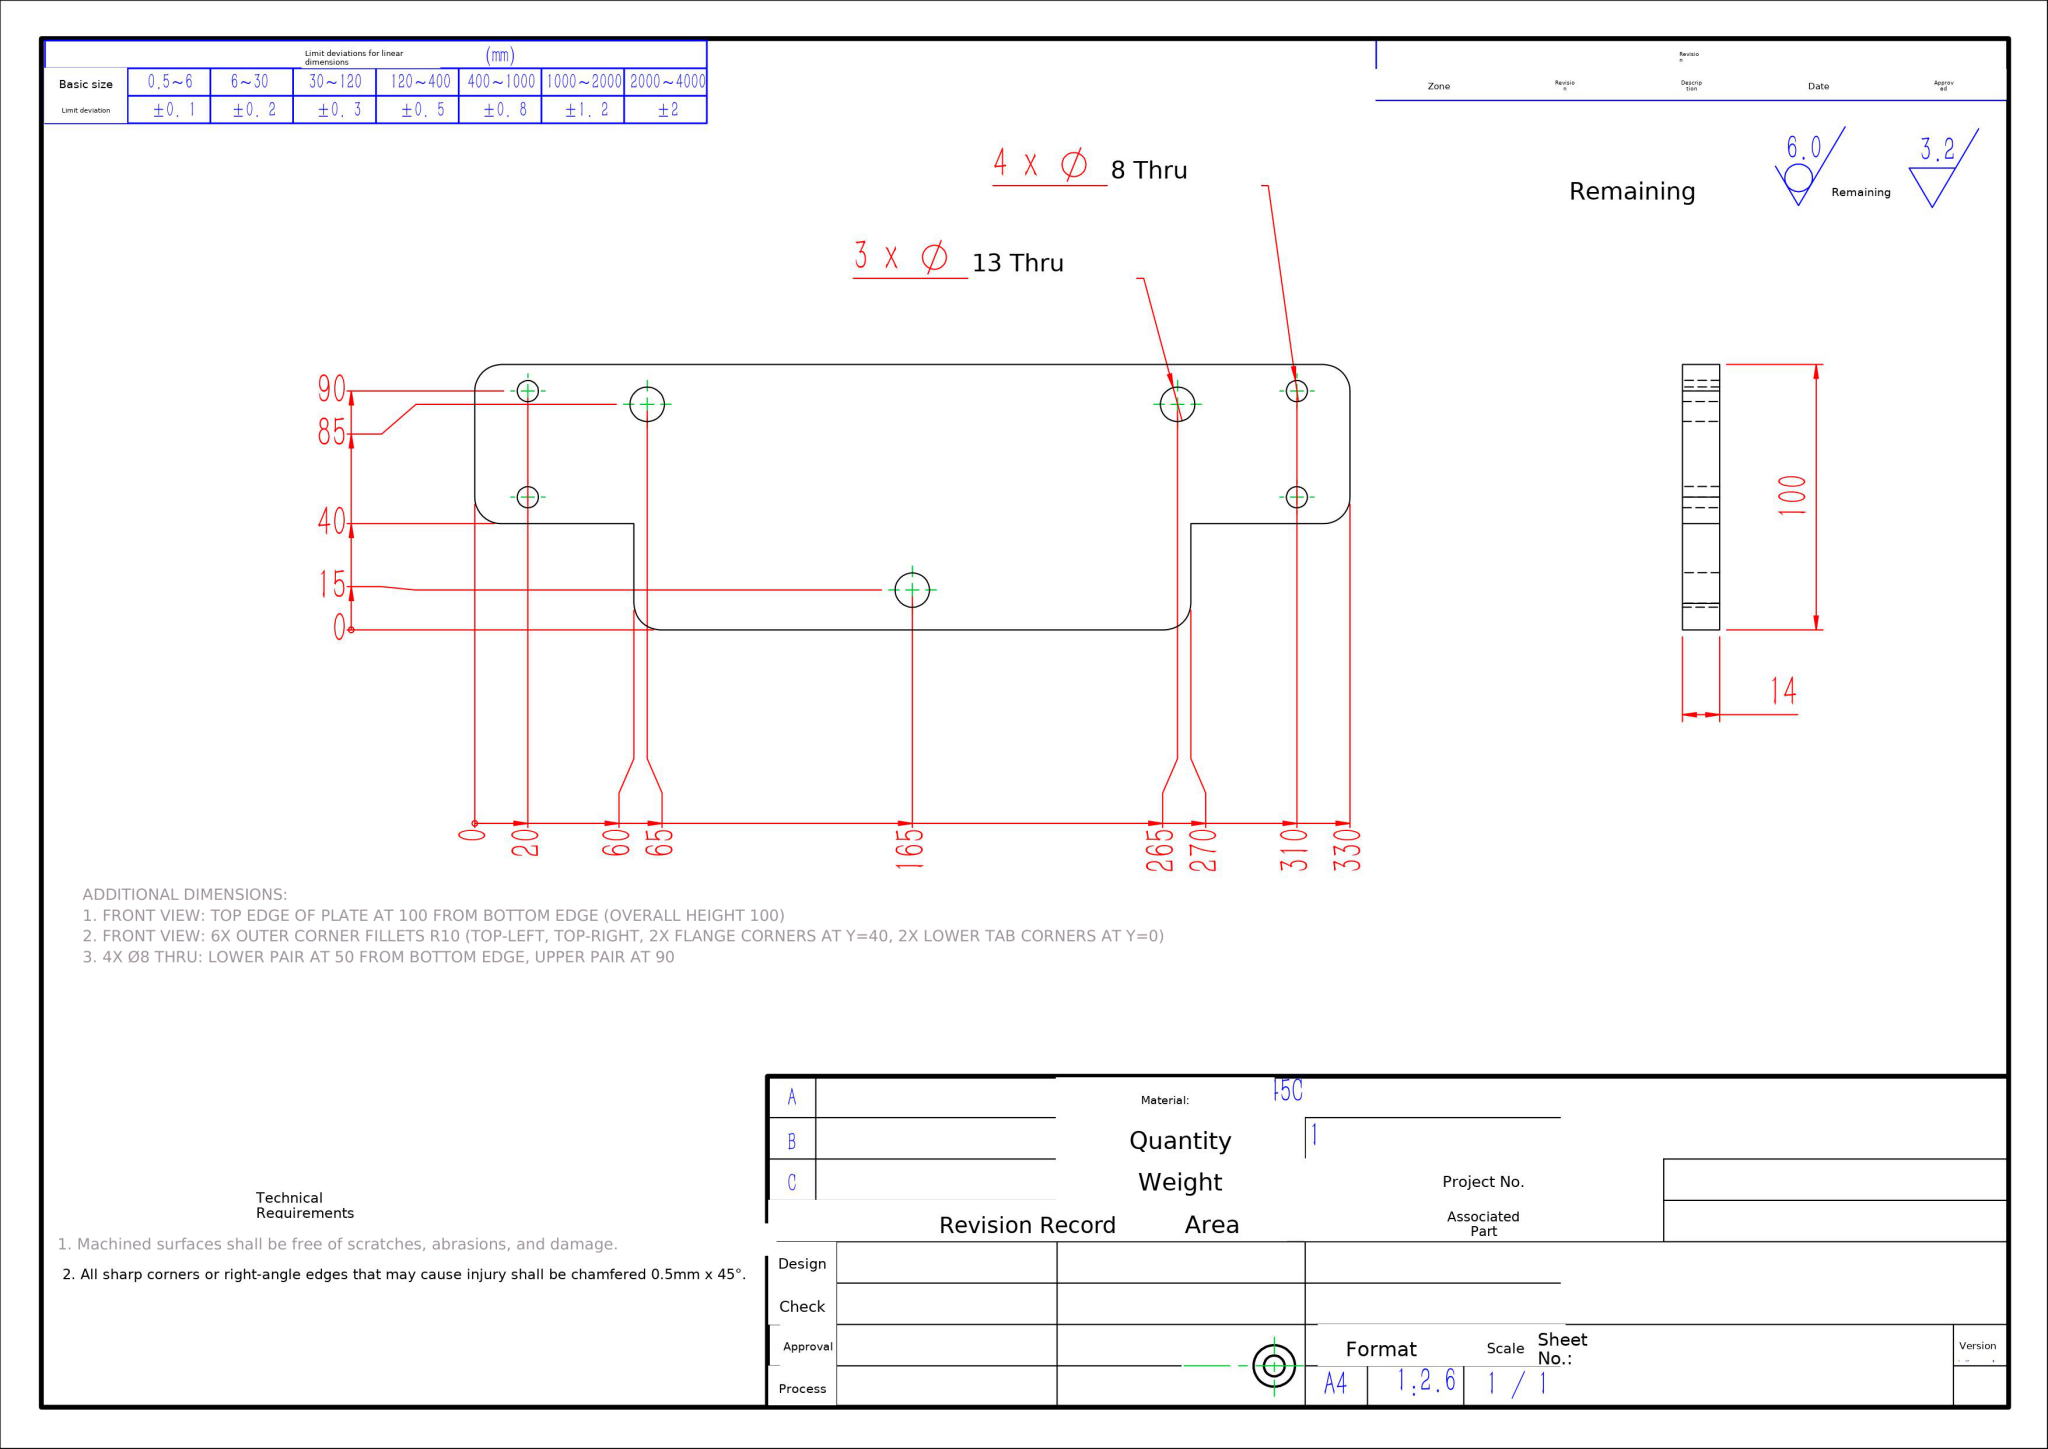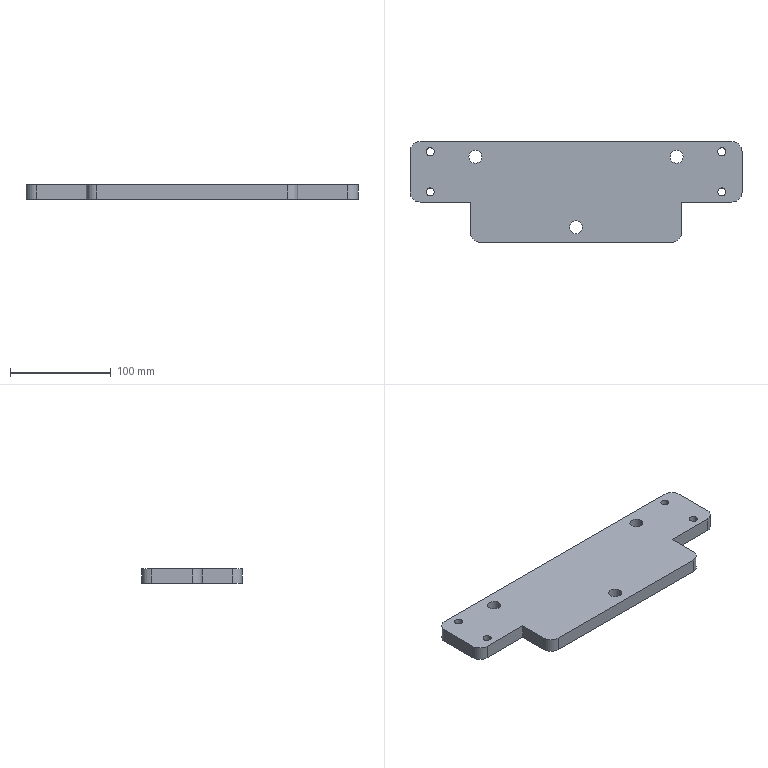Part | NX | mm | 1 solid | 30 faces | box 330 x 100 x 14 mm | volume 384608 mm3 | cylinder 20 | plane 10 | commonest cylinder face diameters 8 x8 13 x6 20 x6
STEP:
#1=COLOUR_RGB('',0.8745,0.,0.1333);
#2=FILL_AREA_STYLE_COLOUR('',#1);
#3=FILL_AREA_STYLE('',(#2));
#4=SURFACE_STYLE_FILL_AREA(#3);
#5=SURFACE_SIDE_STYLE('',(#4));
#6=SURFACE_STYLE_USAGE(.BOTH.,#5);
#7=PRESENTATION_STYLE_ASSIGNMENT((#6));
#8=CARTESIAN_POINT('',(-106.5,35.,0.));
#9=VERTEX_POINT('',#8);
#10=CARTESIAN_POINT('',(-93.5,35.,0.));
#11=VERTEX_POINT('',#10);
#12=CARTESIAN_POINT('',(-100.,35.,0.));
#13=DIRECTION('',(0.,0.,1.));
#14=DIRECTION('',(1.,0.,0.));
#15=AXIS2_PLACEMENT_3D('',#12,#13,#14);
#16=CIRCLE('',#15,6.5);
#17=EDGE_CURVE('',#9,#11,#16,.T.);
#18=ORIENTED_EDGE('',*,*,#17,.F.);
#19=CARTESIAN_POINT('',(-106.5,35.,14.));
#20=VERTEX_POINT('',#19);
#21=CARTESIAN_POINT('',(-106.5,35.,14.));
#22=DIRECTION('',(0.,0.,1.));
#23=VECTOR('',#22,1000.);
#24=LINE('',#21,#23);
#25=EDGE_CURVE('',#9,#20,#24,.T.);
#26=ORIENTED_EDGE('',*,*,#25,.T.);
#27=CARTESIAN_POINT('',(-93.5,35.,14.));
#28=VERTEX_POINT('',#27);
#29=CARTESIAN_POINT('',(-100.,35.,14.));
#30=DIRECTION('',(0.,0.,1.));
#31=DIRECTION('',(1.,0.,0.));
#32=AXIS2_PLACEMENT_3D('',#29,#30,#31);
#33=CIRCLE('',#32,6.5);
#34=EDGE_CURVE('',#20,#28,#33,.T.);
#35=ORIENTED_EDGE('',*,*,#34,.T.);
#36=CARTESIAN_POINT('',(-93.5,35.,14.));
#37=DIRECTION('',(0.,0.,1.));
#38=VECTOR('',#37,1000.);
#39=LINE('',#36,#38);
#40=EDGE_CURVE('',#11,#28,#39,.T.);
#41=ORIENTED_EDGE('',*,*,#40,.F.);
#42=EDGE_LOOP('',(#18,#26,#35,#41));
#43=FACE_OUTER_BOUND('',#42,.T.);
#44=CARTESIAN_POINT('',(-100.,35.,14.));
#45=DIRECTION('',(0.,0.,1.));
#46=DIRECTION('',(1.,0.,0.));
#47=AXIS2_PLACEMENT_3D('',#44,#45,#46);
#48=CYLINDRICAL_SURFACE('',#47,6.5);
#49=ADVANCED_FACE('',(#43),#48,.F.);
#50=CARTESIAN_POINT('',(93.5,35.,0.));
#51=VERTEX_POINT('',#50);
#52=CARTESIAN_POINT('',(106.5,35.,0.));
#53=VERTEX_POINT('',#52);
#54=CARTESIAN_POINT('',(100.,35.,0.));
#55=DIRECTION('',(0.,0.,1.));
#56=DIRECTION('',(1.,0.,0.));
#57=AXIS2_PLACEMENT_3D('',#54,#55,#56);
#58=CIRCLE('',#57,6.5);
#59=EDGE_CURVE('',#51,#53,#58,.T.);
#60=ORIENTED_EDGE('',*,*,#59,.F.);
#61=CARTESIAN_POINT('',(93.5,35.,14.));
#62=VERTEX_POINT('',#61);
#63=CARTESIAN_POINT('',(93.5,35.,14.));
#64=DIRECTION('',(0.,0.,1.));
#65=VECTOR('',#64,1000.);
#66=LINE('',#63,#65);
#67=EDGE_CURVE('',#51,#62,#66,.T.);
#68=ORIENTED_EDGE('',*,*,#67,.T.);
#69=CARTESIAN_POINT('',(106.5,35.,14.));
#70=VERTEX_POINT('',#69);
#71=CARTESIAN_POINT('',(100.,35.,14.));
#72=DIRECTION('',(0.,0.,1.));
#73=DIRECTION('',(1.,0.,0.));
#74=AXIS2_PLACEMENT_3D('',#71,#72,#73);
#75=CIRCLE('',#74,6.5);
#76=EDGE_CURVE('',#62,#70,#75,.T.);
#77=ORIENTED_EDGE('',*,*,#76,.T.);
#78=CARTESIAN_POINT('',(106.5,35.,14.));
#79=DIRECTION('',(0.,0.,1.));
#80=VECTOR('',#79,1000.);
#81=LINE('',#78,#80);
#82=EDGE_CURVE('',#53,#70,#81,.T.);
#83=ORIENTED_EDGE('',*,*,#82,.F.);
#84=EDGE_LOOP('',(#60,#68,#77,#83));
#85=FACE_OUTER_BOUND('',#84,.T.);
#86=CARTESIAN_POINT('',(100.,35.,14.));
#87=DIRECTION('',(0.,0.,1.));
#88=DIRECTION('',(1.,0.,0.));
#89=AXIS2_PLACEMENT_3D('',#86,#87,#88);
#90=CYLINDRICAL_SURFACE('',#89,6.5);
#91=ADVANCED_FACE('',(#85),#90,.F.);
#92=CARTESIAN_POINT('',(-6.5,-35.,0.));
#93=VERTEX_POINT('',#92);
#94=CARTESIAN_POINT('',(6.5,-35.,0.));
#95=VERTEX_POINT('',#94);
#96=CARTESIAN_POINT('',(-0.,-35.,0.));
#97=DIRECTION('',(0.,0.,1.));
#98=DIRECTION('',(1.,0.,0.));
#99=AXIS2_PLACEMENT_3D('',#96,#97,#98);
#100=CIRCLE('',#99,6.5);
#101=EDGE_CURVE('',#93,#95,#100,.T.);
#102=ORIENTED_EDGE('',*,*,#101,.F.);
#103=CARTESIAN_POINT('',(-6.5,-35.,14.));
#104=VERTEX_POINT('',#103);
#105=CARTESIAN_POINT('',(-6.5,-35.,14.));
#106=DIRECTION('',(0.,0.,1.));
#107=VECTOR('',#106,1000.);
#108=LINE('',#105,#107);
#109=EDGE_CURVE('',#93,#104,#108,.T.);
#110=ORIENTED_EDGE('',*,*,#109,.T.);
#111=CARTESIAN_POINT('',(6.5,-35.,14.));
#112=VERTEX_POINT('',#111);
#113=CARTESIAN_POINT('',(-0.,-35.,14.));
#114=DIRECTION('',(0.,0.,1.));
#115=DIRECTION('',(1.,0.,0.));
#116=AXIS2_PLACEMENT_3D('',#113,#114,#115);
#117=CIRCLE('',#116,6.5);
#118=EDGE_CURVE('',#104,#112,#117,.T.);
#119=ORIENTED_EDGE('',*,*,#118,.T.);
#120=CARTESIAN_POINT('',(6.5,-35.,14.));
#121=DIRECTION('',(0.,0.,1.));
#122=VECTOR('',#121,1000.);
#123=LINE('',#120,#122);
#124=EDGE_CURVE('',#95,#112,#123,.T.);
#125=ORIENTED_EDGE('',*,*,#124,.F.);
#126=EDGE_LOOP('',(#102,#110,#119,#125));
#127=FACE_OUTER_BOUND('',#126,.T.);
#128=CARTESIAN_POINT('',(-0.,-35.,14.));
#129=DIRECTION('',(0.,0.,1.));
#130=DIRECTION('',(1.,0.,0.));
#131=AXIS2_PLACEMENT_3D('',#128,#129,#130);
#132=CYLINDRICAL_SURFACE('',#131,6.5);
#133=ADVANCED_FACE('',(#127),#132,.F.);
#134=CARTESIAN_POINT('',(-149.,40.,0.));
#135=VERTEX_POINT('',#134);
#136=CARTESIAN_POINT('',(-141.,40.,0.));
#137=VERTEX_POINT('',#136);
#138=CARTESIAN_POINT('',(-145.,40.,0.));
#139=DIRECTION('',(0.,0.,1.));
#140=DIRECTION('',(1.,0.,0.));
#141=AXIS2_PLACEMENT_3D('',#138,#139,#140);
#142=CIRCLE('',#141,4.);
#143=EDGE_CURVE('',#135,#137,#142,.T.);
#144=ORIENTED_EDGE('',*,*,#143,.F.);
#145=CARTESIAN_POINT('',(-149.,40.,14.));
#146=VERTEX_POINT('',#145);
#147=CARTESIAN_POINT('',(-149.,40.,14.));
#148=DIRECTION('',(0.,0.,1.));
#149=VECTOR('',#148,1000.);
#150=LINE('',#147,#149);
#151=EDGE_CURVE('',#135,#146,#150,.T.);
#152=ORIENTED_EDGE('',*,*,#151,.T.);
#153=CARTESIAN_POINT('',(-141.,40.,14.));
#154=VERTEX_POINT('',#153);
#155=CARTESIAN_POINT('',(-145.,40.,14.));
#156=DIRECTION('',(0.,0.,1.));
#157=DIRECTION('',(1.,0.,0.));
#158=AXIS2_PLACEMENT_3D('',#155,#156,#157);
#159=CIRCLE('',#158,4.);
#160=EDGE_CURVE('',#146,#154,#159,.T.);
#161=ORIENTED_EDGE('',*,*,#160,.T.);
#162=CARTESIAN_POINT('',(-141.,40.,14.));
#163=DIRECTION('',(0.,0.,1.));
#164=VECTOR('',#163,1000.);
#165=LINE('',#162,#164);
#166=EDGE_CURVE('',#137,#154,#165,.T.);
#167=ORIENTED_EDGE('',*,*,#166,.F.);
#168=EDGE_LOOP('',(#144,#152,#161,#167));
#169=FACE_OUTER_BOUND('',#168,.T.);
#170=CARTESIAN_POINT('',(-145.,40.,14.));
#171=DIRECTION('',(0.,0.,1.));
#172=DIRECTION('',(1.,0.,0.));
#173=AXIS2_PLACEMENT_3D('',#170,#171,#172);
#174=CYLINDRICAL_SURFACE('',#173,4.);
#175=ADVANCED_FACE('',(#169),#174,.F.);
#176=CARTESIAN_POINT('',(141.,40.,0.));
#177=VERTEX_POINT('',#176);
#178=CARTESIAN_POINT('',(149.,40.,0.));
#179=VERTEX_POINT('',#178);
#180=CARTESIAN_POINT('',(145.,40.,0.));
#181=DIRECTION('',(0.,0.,1.));
#182=DIRECTION('',(1.,0.,0.));
#183=AXIS2_PLACEMENT_3D('',#180,#181,#182);
#184=CIRCLE('',#183,4.);
#185=EDGE_CURVE('',#177,#179,#184,.T.);
#186=ORIENTED_EDGE('',*,*,#185,.F.);
#187=CARTESIAN_POINT('',(141.,40.,14.));
#188=VERTEX_POINT('',#187);
#189=CARTESIAN_POINT('',(141.,40.,14.));
#190=DIRECTION('',(0.,0.,1.));
#191=VECTOR('',#190,1000.);
#192=LINE('',#189,#191);
#193=EDGE_CURVE('',#177,#188,#192,.T.);
#194=ORIENTED_EDGE('',*,*,#193,.T.);
#195=CARTESIAN_POINT('',(149.,40.,14.));
#196=VERTEX_POINT('',#195);
#197=CARTESIAN_POINT('',(145.,40.,14.));
#198=DIRECTION('',(0.,0.,1.));
#199=DIRECTION('',(1.,0.,0.));
#200=AXIS2_PLACEMENT_3D('',#197,#198,#199);
#201=CIRCLE('',#200,4.);
#202=EDGE_CURVE('',#188,#196,#201,.T.);
#203=ORIENTED_EDGE('',*,*,#202,.T.);
#204=CARTESIAN_POINT('',(149.,40.,14.));
#205=DIRECTION('',(0.,0.,1.));
#206=VECTOR('',#205,1000.);
#207=LINE('',#204,#206);
#208=EDGE_CURVE('',#179,#196,#207,.T.);
#209=ORIENTED_EDGE('',*,*,#208,.F.);
#210=EDGE_LOOP('',(#186,#194,#203,#209));
#211=FACE_OUTER_BOUND('',#210,.T.);
#212=CARTESIAN_POINT('',(145.,40.,14.));
#213=DIRECTION('',(0.,0.,1.));
#214=DIRECTION('',(1.,0.,0.));
#215=AXIS2_PLACEMENT_3D('',#212,#213,#214);
#216=CYLINDRICAL_SURFACE('',#215,4.);
#217=ADVANCED_FACE('',(#211),#216,.F.);
#218=CARTESIAN_POINT('',(-149.,-0.,0.));
#219=VERTEX_POINT('',#218);
#220=CARTESIAN_POINT('',(-141.,-0.,0.));
#221=VERTEX_POINT('',#220);
#222=CARTESIAN_POINT('',(-145.,-0.,0.));
#223=DIRECTION('',(0.,0.,1.));
#224=DIRECTION('',(1.,0.,0.));
#225=AXIS2_PLACEMENT_3D('',#222,#223,#224);
#226=CIRCLE('',#225,4.);
#227=EDGE_CURVE('',#219,#221,#226,.T.);
#228=ORIENTED_EDGE('',*,*,#227,.F.);
#229=CARTESIAN_POINT('',(-149.,-0.,14.));
#230=VERTEX_POINT('',#229);
#231=CARTESIAN_POINT('',(-149.,-0.,14.));
#232=DIRECTION('',(0.,0.,1.));
#233=VECTOR('',#232,1000.);
#234=LINE('',#231,#233);
#235=EDGE_CURVE('',#219,#230,#234,.T.);
#236=ORIENTED_EDGE('',*,*,#235,.T.);
#237=CARTESIAN_POINT('',(-141.,-0.,14.));
#238=VERTEX_POINT('',#237);
#239=CARTESIAN_POINT('',(-145.,-0.,14.));
#240=DIRECTION('',(0.,0.,1.));
#241=DIRECTION('',(1.,0.,0.));
#242=AXIS2_PLACEMENT_3D('',#239,#240,#241);
#243=CIRCLE('',#242,4.);
#244=EDGE_CURVE('',#230,#238,#243,.T.);
#245=ORIENTED_EDGE('',*,*,#244,.T.);
#246=CARTESIAN_POINT('',(-141.,-0.,14.));
#247=DIRECTION('',(0.,0.,1.));
#248=VECTOR('',#247,1000.);
#249=LINE('',#246,#248);
#250=EDGE_CURVE('',#221,#238,#249,.T.);
#251=ORIENTED_EDGE('',*,*,#250,.F.);
#252=EDGE_LOOP('',(#228,#236,#245,#251));
#253=FACE_OUTER_BOUND('',#252,.T.);
#254=CARTESIAN_POINT('',(-145.,-0.,14.));
#255=DIRECTION('',(0.,0.,1.));
#256=DIRECTION('',(1.,0.,0.));
#257=AXIS2_PLACEMENT_3D('',#254,#255,#256);
#258=CYLINDRICAL_SURFACE('',#257,4.);
#259=ADVANCED_FACE('',(#253),#258,.F.);
#260=CARTESIAN_POINT('',(141.,0.,0.));
#261=VERTEX_POINT('',#260);
#262=CARTESIAN_POINT('',(149.,0.,0.));
#263=VERTEX_POINT('',#262);
#264=CARTESIAN_POINT('',(145.,0.,0.));
#265=DIRECTION('',(0.,0.,1.));
#266=DIRECTION('',(1.,0.,0.));
#267=AXIS2_PLACEMENT_3D('',#264,#265,#266);
#268=CIRCLE('',#267,4.);
#269=EDGE_CURVE('',#261,#263,#268,.T.);
#270=ORIENTED_EDGE('',*,*,#269,.F.);
#271=CARTESIAN_POINT('',(141.,0.,14.));
#272=VERTEX_POINT('',#271);
#273=CARTESIAN_POINT('',(141.,0.,14.));
#274=DIRECTION('',(0.,0.,1.));
#275=VECTOR('',#274,1000.);
#276=LINE('',#273,#275);
#277=EDGE_CURVE('',#261,#272,#276,.T.);
#278=ORIENTED_EDGE('',*,*,#277,.T.);
#279=CARTESIAN_POINT('',(149.,0.,14.));
#280=VERTEX_POINT('',#279);
#281=CARTESIAN_POINT('',(145.,0.,14.));
#282=DIRECTION('',(0.,0.,1.));
#283=DIRECTION('',(1.,0.,0.));
#284=AXIS2_PLACEMENT_3D('',#281,#282,#283);
#285=CIRCLE('',#284,4.);
#286=EDGE_CURVE('',#272,#280,#285,.T.);
#287=ORIENTED_EDGE('',*,*,#286,.T.);
#288=CARTESIAN_POINT('',(149.,0.,14.));
#289=DIRECTION('',(0.,0.,1.));
#290=VECTOR('',#289,1000.);
#291=LINE('',#288,#290);
#292=EDGE_CURVE('',#263,#280,#291,.T.);
#293=ORIENTED_EDGE('',*,*,#292,.F.);
#294=EDGE_LOOP('',(#270,#278,#287,#293));
#295=FACE_OUTER_BOUND('',#294,.T.);
#296=CARTESIAN_POINT('',(145.,0.,14.));
#297=DIRECTION('',(0.,0.,1.));
#298=DIRECTION('',(1.,0.,0.));
#299=AXIS2_PLACEMENT_3D('',#296,#297,#298);
#300=CYLINDRICAL_SURFACE('',#299,4.);
#301=ADVANCED_FACE('',(#295),#300,.F.);
#302=CARTESIAN_POINT('',(165.,0.,0.));
#303=VERTEX_POINT('',#302);
#304=CARTESIAN_POINT('',(165.,40.,0.));
#305=VERTEX_POINT('',#304);
#306=CARTESIAN_POINT('',(165.,-50.,0.));
#307=DIRECTION('',(0.,1.,0.));
#308=VECTOR('',#307,1000.);
#309=LINE('',#306,#308);
#310=EDGE_CURVE('',#303,#305,#309,.T.);
#311=ORIENTED_EDGE('',*,*,#310,.T.);
#312=CARTESIAN_POINT('',(165.,40.,14.));
#313=VERTEX_POINT('',#312);
#314=CARTESIAN_POINT('',(165.,40.,14.));
#315=DIRECTION('',(0.,0.,1.));
#316=VECTOR('',#315,1000.);
#317=LINE('',#314,#316);
#318=EDGE_CURVE('',#305,#313,#317,.T.);
#319=ORIENTED_EDGE('',*,*,#318,.T.);
#320=CARTESIAN_POINT('',(165.,0.,14.));
#321=VERTEX_POINT('',#320);
#322=CARTESIAN_POINT('',(165.,-50.,14.));
#323=DIRECTION('',(0.,1.,0.));
#324=VECTOR('',#323,1000.);
#325=LINE('',#322,#324);
#326=EDGE_CURVE('',#321,#313,#325,.T.);
#327=ORIENTED_EDGE('',*,*,#326,.F.);
#328=CARTESIAN_POINT('',(165.,0.,14.));
#329=DIRECTION('',(0.,0.,-1.));
#330=VECTOR('',#329,1000.);
#331=LINE('',#328,#330);
#332=EDGE_CURVE('',#321,#303,#331,.T.);
#333=ORIENTED_EDGE('',*,*,#332,.T.);
#334=EDGE_LOOP('',(#311,#319,#327,#333));
#335=FACE_OUTER_BOUND('',#334,.T.);
#336=CARTESIAN_POINT('',(165.,-50.,14.));
#337=DIRECTION('',(-1.,0.,0.));
#338=DIRECTION('',(0.,0.,1.));
#339=AXIS2_PLACEMENT_3D('',#336,#337,#338);
#340=PLANE('',#339);
#341=ADVANCED_FACE('',(#335),#340,.F.);
#342=CARTESIAN_POINT('',(155.,50.,14.));
#343=VERTEX_POINT('',#342);
#344=CARTESIAN_POINT('',(-155.,50.,14.));
#345=VERTEX_POINT('',#344);
#346=CARTESIAN_POINT('',(-165.,50.,14.));
#347=DIRECTION('',(-1.,0.,0.));
#348=VECTOR('',#347,1000.);
#349=LINE('',#346,#348);
#350=EDGE_CURVE('',#343,#345,#349,.T.);
#351=ORIENTED_EDGE('',*,*,#350,.F.);
#352=CARTESIAN_POINT('',(155.,50.,0.));
#353=VERTEX_POINT('',#352);
#354=CARTESIAN_POINT('',(155.,50.,14.));
#355=DIRECTION('',(0.,0.,-1.));
#356=VECTOR('',#355,1000.);
#357=LINE('',#354,#356);
#358=EDGE_CURVE('',#343,#353,#357,.T.);
#359=ORIENTED_EDGE('',*,*,#358,.T.);
#360=CARTESIAN_POINT('',(-155.,50.,0.));
#361=VERTEX_POINT('',#360);
#362=CARTESIAN_POINT('',(-165.,50.,0.));
#363=DIRECTION('',(-1.,0.,0.));
#364=VECTOR('',#363,1000.);
#365=LINE('',#362,#364);
#366=EDGE_CURVE('',#353,#361,#365,.T.);
#367=ORIENTED_EDGE('',*,*,#366,.T.);
#368=CARTESIAN_POINT('',(-155.,50.,14.));
#369=DIRECTION('',(0.,0.,1.));
#370=VECTOR('',#369,1000.);
#371=LINE('',#368,#370);
#372=EDGE_CURVE('',#361,#345,#371,.T.);
#373=ORIENTED_EDGE('',*,*,#372,.T.);
#374=EDGE_LOOP('',(#351,#359,#367,#373));
#375=FACE_OUTER_BOUND('',#374,.T.);
#376=CARTESIAN_POINT('',(-165.,50.,14.));
#377=DIRECTION('',(0.,-1.,0.));
#378=DIRECTION('',(0.,0.,-1.));
#379=AXIS2_PLACEMENT_3D('',#376,#377,#378);
#380=PLANE('',#379);
#381=ADVANCED_FACE('',(#375),#380,.F.);
#382=CARTESIAN_POINT('',(-165.,40.,0.));
#383=VERTEX_POINT('',#382);
#384=CARTESIAN_POINT('',(-165.,0.,0.));
#385=VERTEX_POINT('',#384);
#386=CARTESIAN_POINT('',(-165.,-50.,0.));
#387=DIRECTION('',(0.,-1.,0.));
#388=VECTOR('',#387,1000.);
#389=LINE('',#386,#388);
#390=EDGE_CURVE('',#383,#385,#389,.T.);
#391=ORIENTED_EDGE('',*,*,#390,.T.);
#392=CARTESIAN_POINT('',(-165.,0.,14.));
#393=VERTEX_POINT('',#392);
#394=CARTESIAN_POINT('',(-165.,0.,14.));
#395=DIRECTION('',(0.,0.,1.));
#396=VECTOR('',#395,1000.);
#397=LINE('',#394,#396);
#398=EDGE_CURVE('',#385,#393,#397,.T.);
#399=ORIENTED_EDGE('',*,*,#398,.T.);
#400=CARTESIAN_POINT('',(-165.,40.,14.));
#401=VERTEX_POINT('',#400);
#402=CARTESIAN_POINT('',(-165.,-50.,14.));
#403=DIRECTION('',(0.,-1.,0.));
#404=VECTOR('',#403,1000.);
#405=LINE('',#402,#404);
#406=EDGE_CURVE('',#401,#393,#405,.T.);
#407=ORIENTED_EDGE('',*,*,#406,.F.);
#408=CARTESIAN_POINT('',(-165.,40.,14.));
#409=DIRECTION('',(0.,0.,-1.));
#410=VECTOR('',#409,1000.);
#411=LINE('',#408,#410);
#412=EDGE_CURVE('',#401,#383,#411,.T.);
#413=ORIENTED_EDGE('',*,*,#412,.T.);
#414=EDGE_LOOP('',(#391,#399,#407,#413));
#415=FACE_OUTER_BOUND('',#414,.T.);
#416=CARTESIAN_POINT('',(-165.,-50.,14.));
#417=DIRECTION('',(1.,0.,0.));
#418=DIRECTION('',(0.,0.,-1.));
#419=AXIS2_PLACEMENT_3D('',#416,#417,#418);
#420=PLANE('',#419);
#421=ADVANCED_FACE('',(#415),#420,.F.);
#422=CARTESIAN_POINT('',(-95.,-50.,0.));
#423=VERTEX_POINT('',#422);
#424=CARTESIAN_POINT('',(95.,-50.,0.));
#425=VERTEX_POINT('',#424);
#426=CARTESIAN_POINT('',(-165.,-50.,0.));
#427=DIRECTION('',(1.,0.,0.));
#428=VECTOR('',#427,1000.);
#429=LINE('',#426,#428);
#430=EDGE_CURVE('',#423,#425,#429,.T.);
#431=ORIENTED_EDGE('',*,*,#430,.T.);
#432=CARTESIAN_POINT('',(95.,-50.,14.));
#433=VERTEX_POINT('',#432);
#434=CARTESIAN_POINT('',(95.,-50.,14.));
#435=DIRECTION('',(0.,0.,1.));
#436=VECTOR('',#435,1000.);
#437=LINE('',#434,#436);
#438=EDGE_CURVE('',#425,#433,#437,.T.);
#439=ORIENTED_EDGE('',*,*,#438,.T.);
#440=CARTESIAN_POINT('',(-95.,-50.,14.));
#441=VERTEX_POINT('',#440);
#442=CARTESIAN_POINT('',(-165.,-50.,14.));
#443=DIRECTION('',(1.,0.,0.));
#444=VECTOR('',#443,1000.);
#445=LINE('',#442,#444);
#446=EDGE_CURVE('',#441,#433,#445,.T.);
#447=ORIENTED_EDGE('',*,*,#446,.F.);
#448=CARTESIAN_POINT('',(-95.,-50.,14.));
#449=DIRECTION('',(0.,0.,-1.));
#450=VECTOR('',#449,1000.);
#451=LINE('',#448,#450);
#452=EDGE_CURVE('',#441,#423,#451,.T.);
#453=ORIENTED_EDGE('',*,*,#452,.T.);
#454=EDGE_LOOP('',(#431,#439,#447,#453));
#455=FACE_OUTER_BOUND('',#454,.T.);
#456=CARTESIAN_POINT('',(-165.,-50.,14.));
#457=DIRECTION('',(0.,1.,0.));
#458=DIRECTION('',(0.,0.,1.));
#459=AXIS2_PLACEMENT_3D('',#456,#457,#458);
#460=PLANE('',#459);
#461=ADVANCED_FACE('',(#455),#460,.F.);
#462=CARTESIAN_POINT('',(-100.,35.,14.));
#463=DIRECTION('',(0.,0.,1.));
#464=DIRECTION('',(1.,0.,0.));
#465=AXIS2_PLACEMENT_3D('',#462,#463,#464);
#466=CIRCLE('',#465,6.5);
#467=EDGE_CURVE('',#28,#20,#466,.T.);
#468=ORIENTED_EDGE('',*,*,#467,.F.);
#469=ORIENTED_EDGE('',*,*,#34,.F.);
#470=EDGE_LOOP('',(#468,#469));
#471=FACE_BOUND('',#470,.T.);
#472=CARTESIAN_POINT('',(100.,35.,14.));
#473=DIRECTION('',(0.,0.,1.));
#474=DIRECTION('',(1.,0.,0.));
#475=AXIS2_PLACEMENT_3D('',#472,#473,#474);
#476=CIRCLE('',#475,6.5);
#477=EDGE_CURVE('',#70,#62,#476,.T.);
#478=ORIENTED_EDGE('',*,*,#477,.F.);
#479=ORIENTED_EDGE('',*,*,#76,.F.);
#480=EDGE_LOOP('',(#478,#479));
#481=FACE_BOUND('',#480,.T.);
#482=CARTESIAN_POINT('',(-0.,-35.,14.));
#483=DIRECTION('',(0.,0.,1.));
#484=DIRECTION('',(1.,0.,0.));
#485=AXIS2_PLACEMENT_3D('',#482,#483,#484);
#486=CIRCLE('',#485,6.5);
#487=EDGE_CURVE('',#112,#104,#486,.T.);
#488=ORIENTED_EDGE('',*,*,#487,.F.);
#489=ORIENTED_EDGE('',*,*,#118,.F.);
#490=EDGE_LOOP('',(#488,#489));
#491=FACE_BOUND('',#490,.T.);
#492=CARTESIAN_POINT('',(-145.,40.,14.));
#493=DIRECTION('',(0.,0.,1.));
#494=DIRECTION('',(1.,0.,0.));
#495=AXIS2_PLACEMENT_3D('',#492,#493,#494);
#496=CIRCLE('',#495,4.);
#497=EDGE_CURVE('',#154,#146,#496,.T.);
#498=ORIENTED_EDGE('',*,*,#497,.F.);
#499=ORIENTED_EDGE('',*,*,#160,.F.);
#500=EDGE_LOOP('',(#498,#499));
#501=FACE_BOUND('',#500,.T.);
#502=CARTESIAN_POINT('',(145.,40.,14.));
#503=DIRECTION('',(0.,0.,1.));
#504=DIRECTION('',(1.,0.,0.));
#505=AXIS2_PLACEMENT_3D('',#502,#503,#504);
#506=CIRCLE('',#505,4.);
#507=EDGE_CURVE('',#196,#188,#506,.T.);
#508=ORIENTED_EDGE('',*,*,#507,.F.);
#509=ORIENTED_EDGE('',*,*,#202,.F.);
#510=EDGE_LOOP('',(#508,#509));
#511=FACE_BOUND('',#510,.T.);
#512=CARTESIAN_POINT('',(-145.,-0.,14.));
#513=DIRECTION('',(0.,0.,1.));
#514=DIRECTION('',(1.,0.,0.));
#515=AXIS2_PLACEMENT_3D('',#512,#513,#514);
#516=CIRCLE('',#515,4.);
#517=EDGE_CURVE('',#238,#230,#516,.T.);
#518=ORIENTED_EDGE('',*,*,#517,.F.);
#519=ORIENTED_EDGE('',*,*,#244,.F.);
#520=EDGE_LOOP('',(#518,#519));
#521=FACE_BOUND('',#520,.T.);
#522=CARTESIAN_POINT('',(145.,0.,14.));
#523=DIRECTION('',(0.,0.,1.));
#524=DIRECTION('',(1.,0.,0.));
#525=AXIS2_PLACEMENT_3D('',#522,#523,#524);
#526=CIRCLE('',#525,4.);
#527=EDGE_CURVE('',#280,#272,#526,.T.);
#528=ORIENTED_EDGE('',*,*,#527,.F.);
#529=ORIENTED_EDGE('',*,*,#286,.F.);
#530=EDGE_LOOP('',(#528,#529));
#531=FACE_BOUND('',#530,.T.);
#532=ORIENTED_EDGE('',*,*,#326,.T.);
#533=CARTESIAN_POINT('',(155.,40.,14.));
#534=DIRECTION('',(0.,0.,1.));
#535=DIRECTION('',(-1.,0.,0.));
#536=AXIS2_PLACEMENT_3D('',#533,#534,#535);
#537=CIRCLE('',#536,10.);
#538=EDGE_CURVE('',#313,#343,#537,.T.);
#539=ORIENTED_EDGE('',*,*,#538,.T.);
#540=ORIENTED_EDGE('',*,*,#350,.T.);
#541=CARTESIAN_POINT('',(-155.,40.,14.));
#542=DIRECTION('',(0.,0.,1.));
#543=DIRECTION('',(-1.,0.,0.));
#544=AXIS2_PLACEMENT_3D('',#541,#542,#543);
#545=CIRCLE('',#544,10.);
#546=EDGE_CURVE('',#345,#401,#545,.T.);
#547=ORIENTED_EDGE('',*,*,#546,.T.);
#548=ORIENTED_EDGE('',*,*,#406,.T.);
#549=CARTESIAN_POINT('',(-155.,-10.,14.));
#550=VERTEX_POINT('',#549);
#551=CARTESIAN_POINT('',(-155.,0.,14.));
#552=DIRECTION('',(0.,0.,1.));
#553=DIRECTION('',(-1.,0.,0.));
#554=AXIS2_PLACEMENT_3D('',#551,#552,#553);
#555=CIRCLE('',#554,10.);
#556=EDGE_CURVE('',#393,#550,#555,.T.);
#557=ORIENTED_EDGE('',*,*,#556,.T.);
#558=CARTESIAN_POINT('',(-105.,-10.,14.));
#559=VERTEX_POINT('',#558);
#560=CARTESIAN_POINT('',(-165.,-10.,14.));
#561=DIRECTION('',(-1.,0.,0.));
#562=VECTOR('',#561,1000.);
#563=LINE('',#560,#562);
#564=EDGE_CURVE('',#559,#550,#563,.T.);
#565=ORIENTED_EDGE('',*,*,#564,.F.);
#566=CARTESIAN_POINT('',(-105.,-40.,14.));
#567=VERTEX_POINT('',#566);
#568=CARTESIAN_POINT('',(-105.,-50.,14.));
#569=DIRECTION('',(0.,1.,0.));
#570=VECTOR('',#569,1000.);
#571=LINE('',#568,#570);
#572=EDGE_CURVE('',#567,#559,#571,.T.);
#573=ORIENTED_EDGE('',*,*,#572,.F.);
#574=CARTESIAN_POINT('',(-95.,-40.,14.));
#575=DIRECTION('',(0.,0.,1.));
#576=DIRECTION('',(-1.,0.,0.));
#577=AXIS2_PLACEMENT_3D('',#574,#575,#576);
#578=CIRCLE('',#577,10.);
#579=EDGE_CURVE('',#567,#441,#578,.T.);
#580=ORIENTED_EDGE('',*,*,#579,.T.);
#581=ORIENTED_EDGE('',*,*,#446,.T.);
#582=CARTESIAN_POINT('',(105.,-40.,14.));
#583=VERTEX_POINT('',#582);
#584=CARTESIAN_POINT('',(95.,-40.,14.));
#585=DIRECTION('',(0.,0.,1.));
#586=DIRECTION('',(-1.,0.,0.));
#587=AXIS2_PLACEMENT_3D('',#584,#585,#586);
#588=CIRCLE('',#587,10.);
#589=EDGE_CURVE('',#433,#583,#588,.T.);
#590=ORIENTED_EDGE('',*,*,#589,.T.);
#591=CARTESIAN_POINT('',(105.,-10.,14.));
#592=VERTEX_POINT('',#591);
#593=CARTESIAN_POINT('',(105.,-50.,14.));
#594=DIRECTION('',(0.,-1.,0.));
#595=VECTOR('',#594,1000.);
#596=LINE('',#593,#595);
#597=EDGE_CURVE('',#592,#583,#596,.T.);
#598=ORIENTED_EDGE('',*,*,#597,.F.);
#599=CARTESIAN_POINT('',(155.,-10.,14.));
#600=VERTEX_POINT('',#599);
#601=CARTESIAN_POINT('',(165.,-10.,14.));
#602=DIRECTION('',(-1.,0.,0.));
#603=VECTOR('',#602,1000.);
#604=LINE('',#601,#603);
#605=EDGE_CURVE('',#600,#592,#604,.T.);
#606=ORIENTED_EDGE('',*,*,#605,.F.);
#607=CARTESIAN_POINT('',(155.,0.,14.));
#608=DIRECTION('',(0.,0.,1.));
#609=DIRECTION('',(-1.,0.,0.));
#610=AXIS2_PLACEMENT_3D('',#607,#608,#609);
#611=CIRCLE('',#610,10.);
#612=EDGE_CURVE('',#600,#321,#611,.T.);
#613=ORIENTED_EDGE('',*,*,#612,.T.);
#614=EDGE_LOOP('',(#532,#539,#540,#547,#548,#557,#565,#573,#580,#581,#590,#598,#606,#613));
#615=FACE_OUTER_BOUND('',#614,.T.);
#616=CARTESIAN_POINT('',(0.,0.,14.));
#617=DIRECTION('',(0.,0.,-1.));
#618=DIRECTION('',(-1.,0.,0.));
#619=AXIS2_PLACEMENT_3D('',#616,#617,#618);
#620=PLANE('',#619);
#621=ADVANCED_FACE('',(#471,#481,#491,#501,#511,#521,#531,#615),#620,.F.);
#622=CARTESIAN_POINT('',(-100.,35.,0.));
#623=DIRECTION('',(0.,0.,1.));
#624=DIRECTION('',(1.,0.,0.));
#625=AXIS2_PLACEMENT_3D('',#622,#623,#624);
#626=CIRCLE('',#625,6.5);
#627=EDGE_CURVE('',#11,#9,#626,.T.);
#628=ORIENTED_EDGE('',*,*,#627,.T.);
#629=ORIENTED_EDGE('',*,*,#17,.T.);
#630=EDGE_LOOP('',(#628,#629));
#631=FACE_BOUND('',#630,.T.);
#632=CARTESIAN_POINT('',(100.,35.,0.));
#633=DIRECTION('',(0.,0.,1.));
#634=DIRECTION('',(1.,0.,0.));
#635=AXIS2_PLACEMENT_3D('',#632,#633,#634);
#636=CIRCLE('',#635,6.5);
#637=EDGE_CURVE('',#53,#51,#636,.T.);
#638=ORIENTED_EDGE('',*,*,#637,.T.);
#639=ORIENTED_EDGE('',*,*,#59,.T.);
#640=EDGE_LOOP('',(#638,#639));
#641=FACE_BOUND('',#640,.T.);
#642=CARTESIAN_POINT('',(-0.,-35.,0.));
#643=DIRECTION('',(0.,0.,1.));
#644=DIRECTION('',(1.,0.,0.));
#645=AXIS2_PLACEMENT_3D('',#642,#643,#644);
#646=CIRCLE('',#645,6.5);
#647=EDGE_CURVE('',#95,#93,#646,.T.);
#648=ORIENTED_EDGE('',*,*,#647,.T.);
#649=ORIENTED_EDGE('',*,*,#101,.T.);
#650=EDGE_LOOP('',(#648,#649));
#651=FACE_BOUND('',#650,.T.);
#652=CARTESIAN_POINT('',(-145.,40.,0.));
#653=DIRECTION('',(0.,0.,1.));
#654=DIRECTION('',(1.,0.,0.));
#655=AXIS2_PLACEMENT_3D('',#652,#653,#654);
#656=CIRCLE('',#655,4.);
#657=EDGE_CURVE('',#137,#135,#656,.T.);
#658=ORIENTED_EDGE('',*,*,#657,.T.);
#659=ORIENTED_EDGE('',*,*,#143,.T.);
#660=EDGE_LOOP('',(#658,#659));
#661=FACE_BOUND('',#660,.T.);
#662=CARTESIAN_POINT('',(145.,40.,0.));
#663=DIRECTION('',(0.,0.,1.));
#664=DIRECTION('',(1.,0.,0.));
#665=AXIS2_PLACEMENT_3D('',#662,#663,#664);
#666=CIRCLE('',#665,4.);
#667=EDGE_CURVE('',#179,#177,#666,.T.);
#668=ORIENTED_EDGE('',*,*,#667,.T.);
#669=ORIENTED_EDGE('',*,*,#185,.T.);
#670=EDGE_LOOP('',(#668,#669));
#671=FACE_BOUND('',#670,.T.);
#672=CARTESIAN_POINT('',(-145.,-0.,0.));
#673=DIRECTION('',(0.,0.,1.));
#674=DIRECTION('',(1.,0.,0.));
#675=AXIS2_PLACEMENT_3D('',#672,#673,#674);
#676=CIRCLE('',#675,4.);
#677=EDGE_CURVE('',#221,#219,#676,.T.);
#678=ORIENTED_EDGE('',*,*,#677,.T.);
#679=ORIENTED_EDGE('',*,*,#227,.T.);
#680=EDGE_LOOP('',(#678,#679));
#681=FACE_BOUND('',#680,.T.);
#682=CARTESIAN_POINT('',(145.,0.,0.));
#683=DIRECTION('',(0.,0.,1.));
#684=DIRECTION('',(1.,0.,0.));
#685=AXIS2_PLACEMENT_3D('',#682,#683,#684);
#686=CIRCLE('',#685,4.);
#687=EDGE_CURVE('',#263,#261,#686,.T.);
#688=ORIENTED_EDGE('',*,*,#687,.T.);
#689=ORIENTED_EDGE('',*,*,#269,.T.);
#690=EDGE_LOOP('',(#688,#689));
#691=FACE_BOUND('',#690,.T.);
#692=ORIENTED_EDGE('',*,*,#366,.F.);
#693=CARTESIAN_POINT('',(155.,40.,0.));
#694=DIRECTION('',(0.,0.,-1.));
#695=DIRECTION('',(-1.,0.,0.));
#696=AXIS2_PLACEMENT_3D('',#693,#694,#695);
#697=CIRCLE('',#696,10.);
#698=EDGE_CURVE('',#353,#305,#697,.T.);
#699=ORIENTED_EDGE('',*,*,#698,.T.);
#700=ORIENTED_EDGE('',*,*,#310,.F.);
#701=CARTESIAN_POINT('',(155.,-10.,0.));
#702=VERTEX_POINT('',#701);
#703=CARTESIAN_POINT('',(155.,0.,0.));
#704=DIRECTION('',(0.,0.,-1.));
#705=DIRECTION('',(-1.,0.,0.));
#706=AXIS2_PLACEMENT_3D('',#703,#704,#705);
#707=CIRCLE('',#706,10.);
#708=EDGE_CURVE('',#303,#702,#707,.T.);
#709=ORIENTED_EDGE('',*,*,#708,.T.);
#710=CARTESIAN_POINT('',(105.,-10.,0.));
#711=VERTEX_POINT('',#710);
#712=CARTESIAN_POINT('',(165.,-10.,0.));
#713=DIRECTION('',(-1.,0.,0.));
#714=VECTOR('',#713,1000.);
#715=LINE('',#712,#714);
#716=EDGE_CURVE('',#702,#711,#715,.T.);
#717=ORIENTED_EDGE('',*,*,#716,.T.);
#718=CARTESIAN_POINT('',(105.,-40.,0.));
#719=VERTEX_POINT('',#718);
#720=CARTESIAN_POINT('',(105.,-50.,0.));
#721=DIRECTION('',(0.,-1.,0.));
#722=VECTOR('',#721,1000.);
#723=LINE('',#720,#722);
#724=EDGE_CURVE('',#711,#719,#723,.T.);
#725=ORIENTED_EDGE('',*,*,#724,.T.);
#726=CARTESIAN_POINT('',(95.,-40.,0.));
#727=DIRECTION('',(0.,0.,-1.));
#728=DIRECTION('',(-1.,0.,0.));
#729=AXIS2_PLACEMENT_3D('',#726,#727,#728);
#730=CIRCLE('',#729,10.);
#731=EDGE_CURVE('',#719,#425,#730,.T.);
#732=ORIENTED_EDGE('',*,*,#731,.T.);
#733=ORIENTED_EDGE('',*,*,#430,.F.);
#734=CARTESIAN_POINT('',(-105.,-40.,0.));
#735=VERTEX_POINT('',#734);
#736=CARTESIAN_POINT('',(-95.,-40.,0.));
#737=DIRECTION('',(0.,0.,-1.));
#738=DIRECTION('',(-1.,0.,0.));
#739=AXIS2_PLACEMENT_3D('',#736,#737,#738);
#740=CIRCLE('',#739,10.);
#741=EDGE_CURVE('',#423,#735,#740,.T.);
#742=ORIENTED_EDGE('',*,*,#741,.T.);
#743=CARTESIAN_POINT('',(-105.,-10.,0.));
#744=VERTEX_POINT('',#743);
#745=CARTESIAN_POINT('',(-105.,-50.,0.));
#746=DIRECTION('',(0.,1.,0.));
#747=VECTOR('',#746,1000.);
#748=LINE('',#745,#747);
#749=EDGE_CURVE('',#735,#744,#748,.T.);
#750=ORIENTED_EDGE('',*,*,#749,.T.);
#751=CARTESIAN_POINT('',(-155.,-10.,0.));
#752=VERTEX_POINT('',#751);
#753=CARTESIAN_POINT('',(-165.,-10.,0.));
#754=DIRECTION('',(-1.,0.,0.));
#755=VECTOR('',#754,1000.);
#756=LINE('',#753,#755);
#757=EDGE_CURVE('',#744,#752,#756,.T.);
#758=ORIENTED_EDGE('',*,*,#757,.T.);
#759=CARTESIAN_POINT('',(-155.,0.,0.));
#760=DIRECTION('',(0.,0.,-1.));
#761=DIRECTION('',(-1.,0.,0.));
#762=AXIS2_PLACEMENT_3D('',#759,#760,#761);
#763=CIRCLE('',#762,10.);
#764=EDGE_CURVE('',#752,#385,#763,.T.);
#765=ORIENTED_EDGE('',*,*,#764,.T.);
#766=ORIENTED_EDGE('',*,*,#390,.F.);
#767=CARTESIAN_POINT('',(-155.,40.,0.));
#768=DIRECTION('',(0.,0.,-1.));
#769=DIRECTION('',(-1.,0.,0.));
#770=AXIS2_PLACEMENT_3D('',#767,#768,#769);
#771=CIRCLE('',#770,10.);
#772=EDGE_CURVE('',#383,#361,#771,.T.);
#773=ORIENTED_EDGE('',*,*,#772,.T.);
#774=EDGE_LOOP('',(#692,#699,#700,#709,#717,#725,#732,#733,#742,#750,#758,#765,#766,#773));
#775=FACE_OUTER_BOUND('',#774,.T.);
#776=CARTESIAN_POINT('',(0.,0.,0.));
#777=DIRECTION('',(0.,0.,-1.));
#778=DIRECTION('',(-1.,0.,0.));
#779=AXIS2_PLACEMENT_3D('',#776,#777,#778);
#780=PLANE('',#779);
#781=ADVANCED_FACE('',(#631,#641,#651,#661,#671,#681,#691,#775),#780,.T.);
#782=ORIENTED_EDGE('',*,*,#597,.T.);
#783=CARTESIAN_POINT('',(105.,-40.,0.));
#784=DIRECTION('',(0.,0.,-1.));
#785=VECTOR('',#784,1000.);
#786=LINE('',#783,#785);
#787=EDGE_CURVE('',#583,#719,#786,.T.);
#788=ORIENTED_EDGE('',*,*,#787,.T.);
#789=ORIENTED_EDGE('',*,*,#724,.F.);
#790=CARTESIAN_POINT('',(105.,-10.,0.));
#791=DIRECTION('',(0.,0.,1.));
#792=VECTOR('',#791,1000.);
#793=LINE('',#790,#792);
#794=EDGE_CURVE('',#711,#592,#793,.T.);
#795=ORIENTED_EDGE('',*,*,#794,.T.);
#796=EDGE_LOOP('',(#782,#788,#789,#795));
#797=FACE_OUTER_BOUND('',#796,.T.);
#798=CARTESIAN_POINT('',(105.,-50.,0.));
#799=DIRECTION('',(-1.,0.,0.));
#800=DIRECTION('',(0.,0.,1.));
#801=AXIS2_PLACEMENT_3D('',#798,#799,#800);
#802=PLANE('',#801);
#803=ADVANCED_FACE('',(#797),#802,.F.);
#804=ORIENTED_EDGE('',*,*,#716,.F.);
#805=CARTESIAN_POINT('',(155.,-10.,0.));
#806=DIRECTION('',(0.,0.,1.));
#807=VECTOR('',#806,1000.);
#808=LINE('',#805,#807);
#809=EDGE_CURVE('',#702,#600,#808,.T.);
#810=ORIENTED_EDGE('',*,*,#809,.T.);
#811=ORIENTED_EDGE('',*,*,#605,.T.);
#812=ORIENTED_EDGE('',*,*,#794,.F.);
#813=EDGE_LOOP('',(#804,#810,#811,#812));
#814=FACE_OUTER_BOUND('',#813,.T.);
#815=CARTESIAN_POINT('',(165.,-10.,0.));
#816=DIRECTION('',(0.,1.,0.));
#817=DIRECTION('',(0.,0.,1.));
#818=AXIS2_PLACEMENT_3D('',#815,#816,#817);
#819=PLANE('',#818);
#820=ADVANCED_FACE('',(#814),#819,.F.);
#821=ORIENTED_EDGE('',*,*,#564,.T.);
#822=CARTESIAN_POINT('',(-155.,-10.,0.));
#823=DIRECTION('',(0.,0.,-1.));
#824=VECTOR('',#823,1000.);
#825=LINE('',#822,#824);
#826=EDGE_CURVE('',#550,#752,#825,.T.);
#827=ORIENTED_EDGE('',*,*,#826,.T.);
#828=ORIENTED_EDGE('',*,*,#757,.F.);
#829=CARTESIAN_POINT('',(-105.,-10.,0.));
#830=DIRECTION('',(0.,0.,1.));
#831=VECTOR('',#830,1000.);
#832=LINE('',#829,#831);
#833=EDGE_CURVE('',#744,#559,#832,.T.);
#834=ORIENTED_EDGE('',*,*,#833,.T.);
#835=EDGE_LOOP('',(#821,#827,#828,#834));
#836=FACE_OUTER_BOUND('',#835,.T.);
#837=CARTESIAN_POINT('',(-165.,-10.,0.));
#838=DIRECTION('',(0.,1.,0.));
#839=DIRECTION('',(0.,0.,1.));
#840=AXIS2_PLACEMENT_3D('',#837,#838,#839);
#841=PLANE('',#840);
#842=ADVANCED_FACE('',(#836),#841,.F.);
#843=ORIENTED_EDGE('',*,*,#749,.F.);
#844=CARTESIAN_POINT('',(-105.,-40.,0.));
#845=DIRECTION('',(0.,0.,1.));
#846=VECTOR('',#845,1000.);
#847=LINE('',#844,#846);
#848=EDGE_CURVE('',#735,#567,#847,.T.);
#849=ORIENTED_EDGE('',*,*,#848,.T.);
#850=ORIENTED_EDGE('',*,*,#572,.T.);
#851=ORIENTED_EDGE('',*,*,#833,.F.);
#852=EDGE_LOOP('',(#843,#849,#850,#851));
#853=FACE_OUTER_BOUND('',#852,.T.);
#854=CARTESIAN_POINT('',(-105.,-50.,0.));
#855=DIRECTION('',(1.,0.,0.));
#856=DIRECTION('',(0.,0.,-1.));
#857=AXIS2_PLACEMENT_3D('',#854,#855,#856);
#858=PLANE('',#857);
#859=ADVANCED_FACE('',(#853),#858,.F.);
#860=ORIENTED_EDGE('',*,*,#538,.F.);
#861=ORIENTED_EDGE('',*,*,#318,.F.);
#862=ORIENTED_EDGE('',*,*,#698,.F.);
#863=ORIENTED_EDGE('',*,*,#358,.F.);
#864=EDGE_LOOP('',(#860,#861,#862,#863));
#865=FACE_OUTER_BOUND('',#864,.T.);
#866=CARTESIAN_POINT('',(155.,40.,14.));
#867=DIRECTION('',(0.,0.,-1.));
#868=DIRECTION('',(-1.,0.,0.));
#869=AXIS2_PLACEMENT_3D('',#866,#867,#868);
#870=CYLINDRICAL_SURFACE('',#869,10.);
#871=ADVANCED_FACE('',(#865),#870,.T.);
#872=ORIENTED_EDGE('',*,*,#708,.F.);
#873=ORIENTED_EDGE('',*,*,#332,.F.);
#874=ORIENTED_EDGE('',*,*,#612,.F.);
#875=ORIENTED_EDGE('',*,*,#809,.F.);
#876=EDGE_LOOP('',(#872,#873,#874,#875));
#877=FACE_OUTER_BOUND('',#876,.T.);
#878=CARTESIAN_POINT('',(155.,0.,0.));
#879=DIRECTION('',(0.,0.,1.));
#880=DIRECTION('',(1.,0.,0.));
#881=AXIS2_PLACEMENT_3D('',#878,#879,#880);
#882=CYLINDRICAL_SURFACE('',#881,10.);
#883=ADVANCED_FACE('',(#877),#882,.T.);
#884=ORIENTED_EDGE('',*,*,#731,.F.);
#885=ORIENTED_EDGE('',*,*,#787,.F.);
#886=ORIENTED_EDGE('',*,*,#589,.F.);
#887=ORIENTED_EDGE('',*,*,#438,.F.);
#888=EDGE_LOOP('',(#884,#885,#886,#887));
#889=FACE_OUTER_BOUND('',#888,.T.);
#890=CARTESIAN_POINT('',(95.,-40.,14.));
#891=DIRECTION('',(0.,0.,1.));
#892=DIRECTION('',(1.,0.,0.));
#893=AXIS2_PLACEMENT_3D('',#890,#891,#892);
#894=CYLINDRICAL_SURFACE('',#893,10.);
#895=ADVANCED_FACE('',(#889),#894,.T.);
#896=ORIENTED_EDGE('',*,*,#741,.F.);
#897=ORIENTED_EDGE('',*,*,#452,.F.);
#898=ORIENTED_EDGE('',*,*,#579,.F.);
#899=ORIENTED_EDGE('',*,*,#848,.F.);
#900=EDGE_LOOP('',(#896,#897,#898,#899));
#901=FACE_OUTER_BOUND('',#900,.T.);
#902=CARTESIAN_POINT('',(-95.,-40.,0.));
#903=DIRECTION('',(0.,0.,1.));
#904=DIRECTION('',(1.,0.,0.));
#905=AXIS2_PLACEMENT_3D('',#902,#903,#904);
#906=CYLINDRICAL_SURFACE('',#905,10.);
#907=ADVANCED_FACE('',(#901),#906,.T.);
#908=ORIENTED_EDGE('',*,*,#764,.F.);
#909=ORIENTED_EDGE('',*,*,#826,.F.);
#910=ORIENTED_EDGE('',*,*,#556,.F.);
#911=ORIENTED_EDGE('',*,*,#398,.F.);
#912=EDGE_LOOP('',(#908,#909,#910,#911));
#913=FACE_OUTER_BOUND('',#912,.T.);
#914=CARTESIAN_POINT('',(-155.,0.,14.));
#915=DIRECTION('',(0.,0.,1.));
#916=DIRECTION('',(1.,0.,0.));
#917=AXIS2_PLACEMENT_3D('',#914,#915,#916);
#918=CYLINDRICAL_SURFACE('',#917,10.);
#919=ADVANCED_FACE('',(#913),#918,.T.);
#920=ORIENTED_EDGE('',*,*,#546,.F.);
#921=ORIENTED_EDGE('',*,*,#372,.F.);
#922=ORIENTED_EDGE('',*,*,#772,.F.);
#923=ORIENTED_EDGE('',*,*,#412,.F.);
#924=EDGE_LOOP('',(#920,#921,#922,#923));
#925=FACE_OUTER_BOUND('',#924,.T.);
#926=CARTESIAN_POINT('',(-155.,40.,14.));
#927=DIRECTION('',(0.,0.,-1.));
#928=DIRECTION('',(-1.,0.,0.));
#929=AXIS2_PLACEMENT_3D('',#926,#927,#928);
#930=CYLINDRICAL_SURFACE('',#929,10.);
#931=ADVANCED_FACE('',(#925),#930,.T.);
#932=ORIENTED_EDGE('',*,*,#277,.F.);
#933=ORIENTED_EDGE('',*,*,#687,.F.);
#934=ORIENTED_EDGE('',*,*,#292,.T.);
#935=ORIENTED_EDGE('',*,*,#527,.T.);
#936=EDGE_LOOP('',(#932,#933,#934,#935));
#937=FACE_OUTER_BOUND('',#936,.T.);
#938=CARTESIAN_POINT('',(145.,0.,14.));
#939=DIRECTION('',(0.,0.,1.));
#940=DIRECTION('',(1.,0.,0.));
#941=AXIS2_PLACEMENT_3D('',#938,#939,#940);
#942=CYLINDRICAL_SURFACE('',#941,4.);
#943=ADVANCED_FACE('',(#937),#942,.F.);
#944=ORIENTED_EDGE('',*,*,#235,.F.);
#945=ORIENTED_EDGE('',*,*,#677,.F.);
#946=ORIENTED_EDGE('',*,*,#250,.T.);
#947=ORIENTED_EDGE('',*,*,#517,.T.);
#948=EDGE_LOOP('',(#944,#945,#946,#947));
#949=FACE_OUTER_BOUND('',#948,.T.);
#950=CARTESIAN_POINT('',(-145.,-0.,14.));
#951=DIRECTION('',(0.,0.,1.));
#952=DIRECTION('',(1.,0.,0.));
#953=AXIS2_PLACEMENT_3D('',#950,#951,#952);
#954=CYLINDRICAL_SURFACE('',#953,4.);
#955=ADVANCED_FACE('',(#949),#954,.F.);
#956=ORIENTED_EDGE('',*,*,#193,.F.);
#957=ORIENTED_EDGE('',*,*,#667,.F.);
#958=ORIENTED_EDGE('',*,*,#208,.T.);
#959=ORIENTED_EDGE('',*,*,#507,.T.);
#960=EDGE_LOOP('',(#956,#957,#958,#959));
#961=FACE_OUTER_BOUND('',#960,.T.);
#962=CARTESIAN_POINT('',(145.,40.,14.));
#963=DIRECTION('',(0.,0.,1.));
#964=DIRECTION('',(1.,0.,0.));
#965=AXIS2_PLACEMENT_3D('',#962,#963,#964);
#966=CYLINDRICAL_SURFACE('',#965,4.);
#967=ADVANCED_FACE('',(#961),#966,.F.);
#968=ORIENTED_EDGE('',*,*,#151,.F.);
#969=ORIENTED_EDGE('',*,*,#657,.F.);
#970=ORIENTED_EDGE('',*,*,#166,.T.);
#971=ORIENTED_EDGE('',*,*,#497,.T.);
#972=EDGE_LOOP('',(#968,#969,#970,#971));
#973=FACE_OUTER_BOUND('',#972,.T.);
#974=CARTESIAN_POINT('',(-145.,40.,14.));
#975=DIRECTION('',(0.,0.,1.));
#976=DIRECTION('',(1.,0.,0.));
#977=AXIS2_PLACEMENT_3D('',#974,#975,#976);
#978=CYLINDRICAL_SURFACE('',#977,4.);
#979=ADVANCED_FACE('',(#973),#978,.F.);
#980=ORIENTED_EDGE('',*,*,#109,.F.);
#981=ORIENTED_EDGE('',*,*,#647,.F.);
#982=ORIENTED_EDGE('',*,*,#124,.T.);
#983=ORIENTED_EDGE('',*,*,#487,.T.);
#984=EDGE_LOOP('',(#980,#981,#982,#983));
#985=FACE_OUTER_BOUND('',#984,.T.);
#986=CARTESIAN_POINT('',(-0.,-35.,14.));
#987=DIRECTION('',(0.,0.,1.));
#988=DIRECTION('',(1.,0.,0.));
#989=AXIS2_PLACEMENT_3D('',#986,#987,#988);
#990=CYLINDRICAL_SURFACE('',#989,6.5);
#991=ADVANCED_FACE('',(#985),#990,.F.);
#992=ORIENTED_EDGE('',*,*,#67,.F.);
#993=ORIENTED_EDGE('',*,*,#637,.F.);
#994=ORIENTED_EDGE('',*,*,#82,.T.);
#995=ORIENTED_EDGE('',*,*,#477,.T.);
#996=EDGE_LOOP('',(#992,#993,#994,#995));
#997=FACE_OUTER_BOUND('',#996,.T.);
#998=CARTESIAN_POINT('',(100.,35.,14.));
#999=DIRECTION('',(0.,0.,1.));
#1000=DIRECTION('',(1.,0.,0.));
#1001=AXIS2_PLACEMENT_3D('',#998,#999,#1000);
#1002=CYLINDRICAL_SURFACE('',#1001,6.5);
#1003=ADVANCED_FACE('',(#997),#1002,.F.);
#1004=ORIENTED_EDGE('',*,*,#25,.F.);
#1005=ORIENTED_EDGE('',*,*,#627,.F.);
#1006=ORIENTED_EDGE('',*,*,#40,.T.);
#1007=ORIENTED_EDGE('',*,*,#467,.T.);
#1008=EDGE_LOOP('',(#1004,#1005,#1006,#1007));
#1009=FACE_OUTER_BOUND('',#1008,.T.);
#1010=CARTESIAN_POINT('',(-100.,35.,14.));
#1011=DIRECTION('',(0.,0.,1.));
#1012=DIRECTION('',(1.,0.,0.));
#1013=AXIS2_PLACEMENT_3D('',#1010,#1011,#1012);
#1014=CYLINDRICAL_SURFACE('',#1013,6.5);
#1015=ADVANCED_FACE('',(#1009),#1014,.F.);
#1016=CLOSED_SHELL('',(#49,#91,#133,#175,#217,#259,#301,#341,#381,#421,#461,#621,#781,#803,#820,#842,#859,#871,#883,#895,#907,#919,#931,#943,#955,#967,#979,#991,#1003,#1015));
#1017=MANIFOLD_SOLID_BREP('',#1016);
#1018=STYLED_ITEM('',(#7),#1017);
#1019=(LENGTH_UNIT()NAMED_UNIT(*)SI_UNIT(.MILLI.,.METRE.));
#1020=UNCERTAINTY_MEASURE_WITH_UNIT(LENGTH_MEASURE(0.00001),#1019,'','');
#1021=(NAMED_UNIT(*)PLANE_ANGLE_UNIT()SI_UNIT($,.RADIAN.));
#1022=(NAMED_UNIT(*)SI_UNIT($,.STERADIAN.)SOLID_ANGLE_UNIT());
#1023=(GEOMETRIC_REPRESENTATION_CONTEXT(3)GLOBAL_UNCERTAINTY_ASSIGNED_CONTEXT((#1020))GLOBAL_UNIT_ASSIGNED_CONTEXT((#1019,#1021,#1022))REPRESENTATION_CONTEXT('',''));
#1024=MECHANICAL_DESIGN_GEOMETRIC_PRESENTATION_REPRESENTATION('',(#1018),#1023);
#1025=COLOUR_RGB('',0.8745,0.,0.1333);
#1026=FILL_AREA_STYLE_COLOUR('',#1025);
#1027=FILL_AREA_STYLE('',(#1026));
#1028=SURFACE_STYLE_FILL_AREA(#1027);
#1029=SURFACE_SIDE_STYLE('',(#1028));
#1030=SURFACE_STYLE_USAGE(.BOTH.,#1029);
#1031=PRESENTATION_STYLE_ASSIGNMENT((#1030));
#1032=CARTESIAN_POINT('',(0.,0.,0.));
#1033=DIRECTION('',(0.,0.,1.));
#1034=DIRECTION('',(1.,0.,0.));
#1035=AXIS2_PLACEMENT_3D('',#1032,#1033,#1034);
#1036=(LENGTH_UNIT()NAMED_UNIT(*)SI_UNIT(.MILLI.,.METRE.));
#1037=UNCERTAINTY_MEASURE_WITH_UNIT(LENGTH_MEASURE(0.00001),#1036,'','');
#1038=(NAMED_UNIT(*)PLANE_ANGLE_UNIT()SI_UNIT($,.RADIAN.));
#1039=(NAMED_UNIT(*)SI_UNIT($,.STERADIAN.)SOLID_ANGLE_UNIT());
#1040=(GEOMETRIC_REPRESENTATION_CONTEXT(3)GLOBAL_UNCERTAINTY_ASSIGNED_CONTEXT((#1037))GLOBAL_UNIT_ASSIGNED_CONTEXT((#1036,#1038,#1039))REPRESENTATION_CONTEXT('',''));
#1041=ADVANCED_BREP_SHAPE_REPRESENTATION('',(#1017,#1035),#1040);
#1042=STYLED_ITEM('',(#1031),#1041);
#1043=PRESENTATION_LAYER_ASSIGNMENT('','',(#1042));
#1044=PRESENTATION_LAYER_ASSIGNMENT('','',(#1018));
#1045=(LENGTH_UNIT()NAMED_UNIT(*)SI_UNIT(.MILLI.,.METRE.));
#1046=UNCERTAINTY_MEASURE_WITH_UNIT(LENGTH_MEASURE(0.00001),#1045,'','');
#1047=(NAMED_UNIT(*)PLANE_ANGLE_UNIT()SI_UNIT($,.RADIAN.));
#1048=(NAMED_UNIT(*)SI_UNIT($,.STERADIAN.)SOLID_ANGLE_UNIT());
#1049=(GEOMETRIC_REPRESENTATION_CONTEXT(3)GLOBAL_UNCERTAINTY_ASSIGNED_CONTEXT((#1046))GLOBAL_UNIT_ASSIGNED_CONTEXT((#1045,#1047,#1048))REPRESENTATION_CONTEXT('',''));
#1050=MECHANICAL_DESIGN_GEOMETRIC_PRESENTATION_REPRESENTATION('',(#1042),#1049);